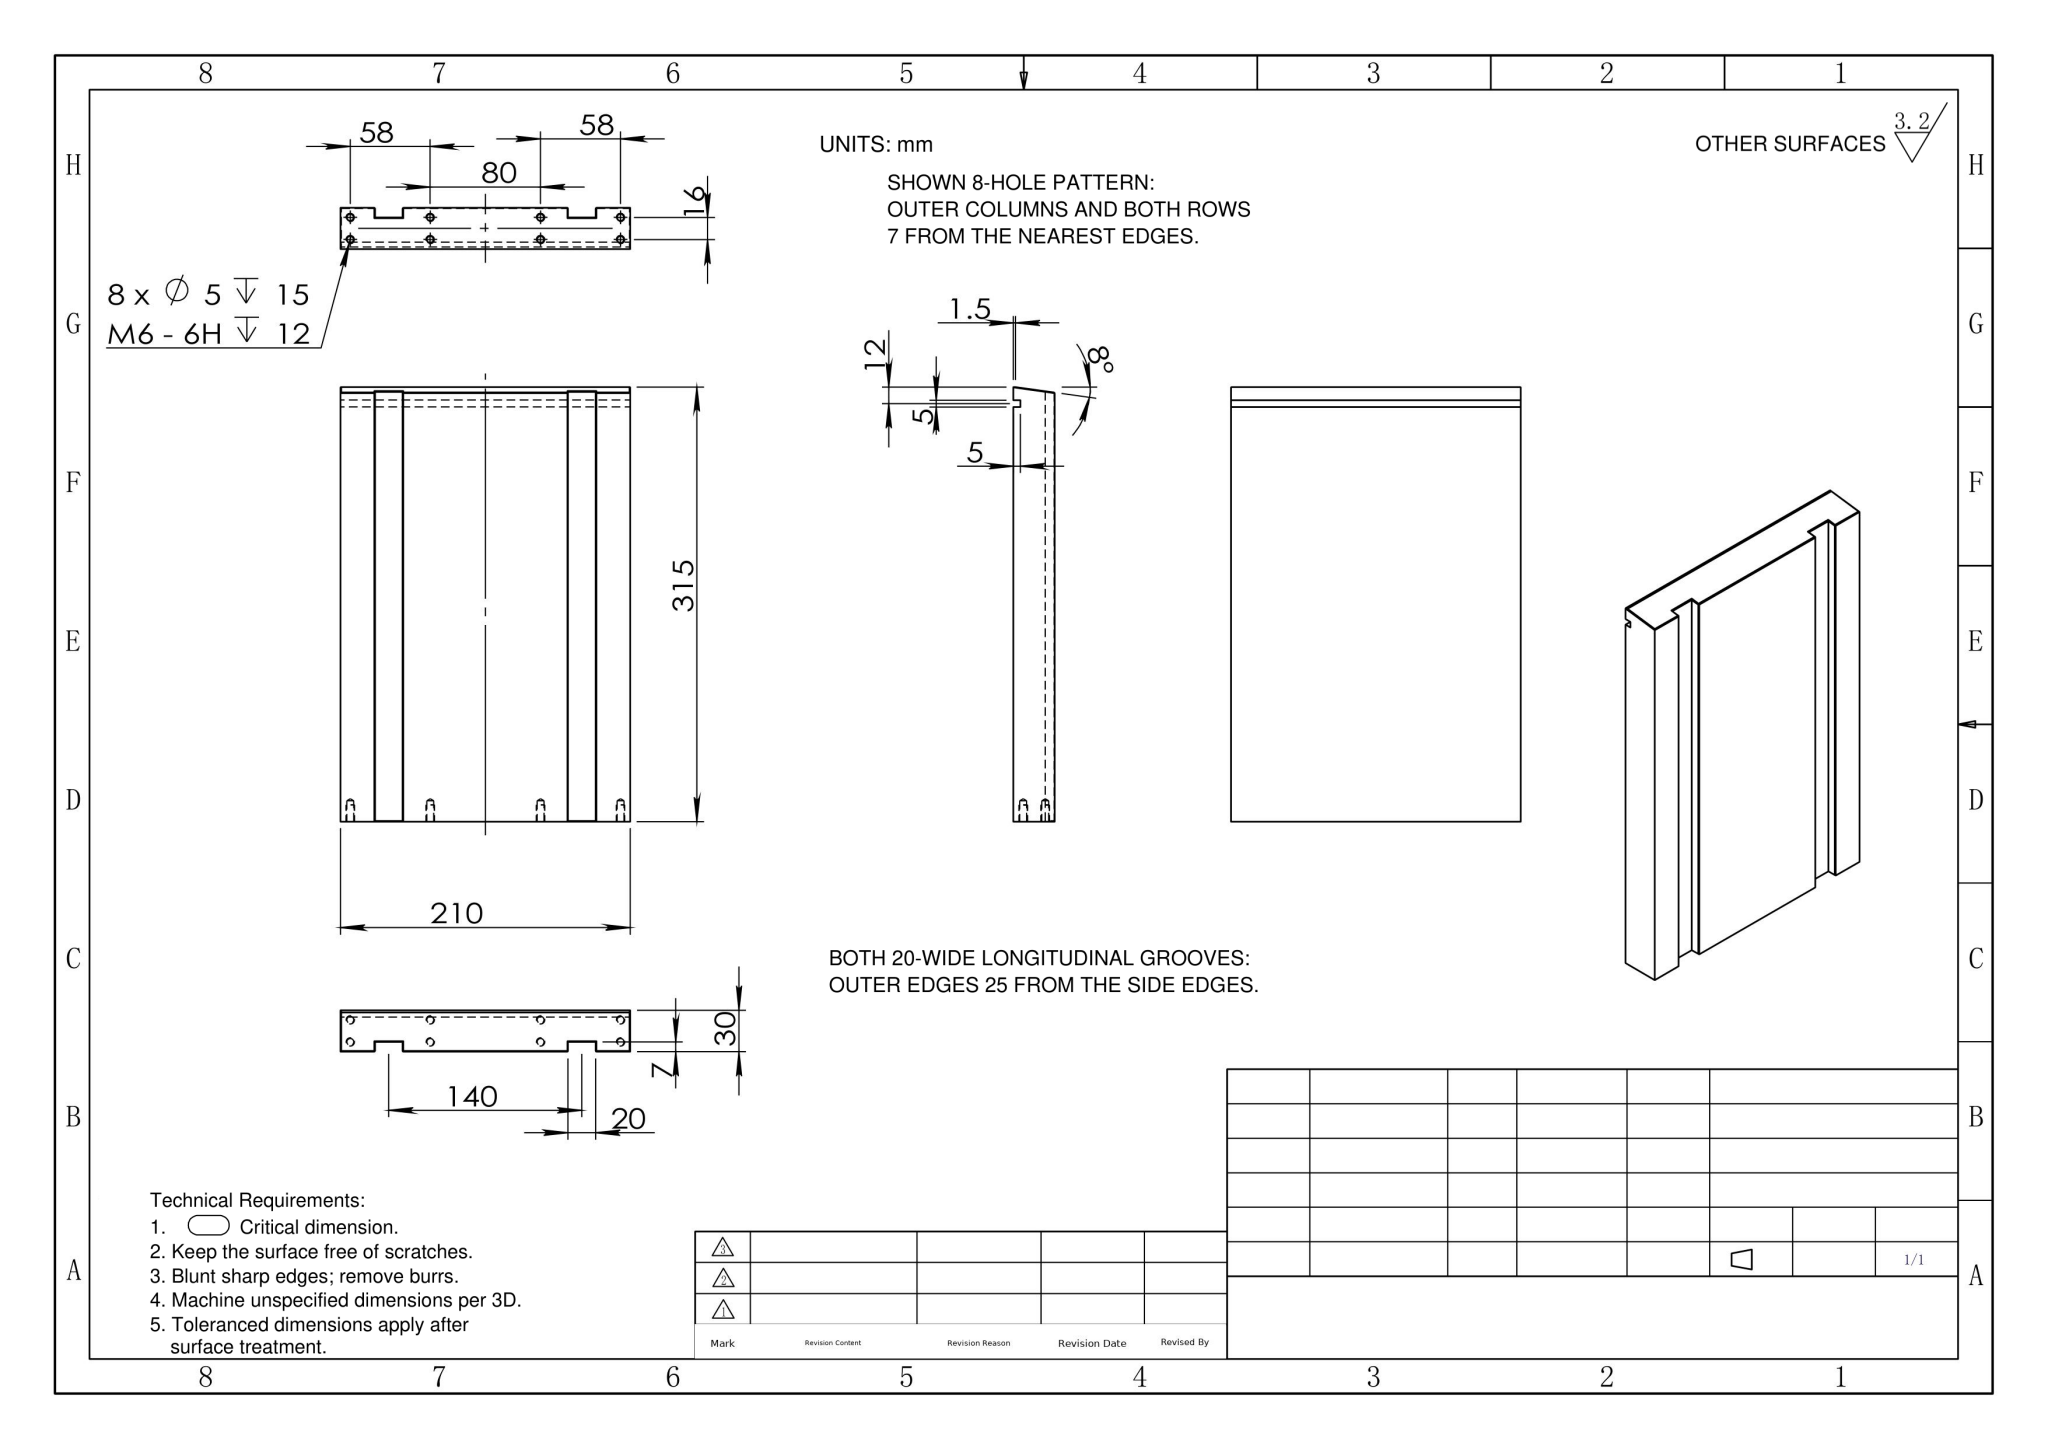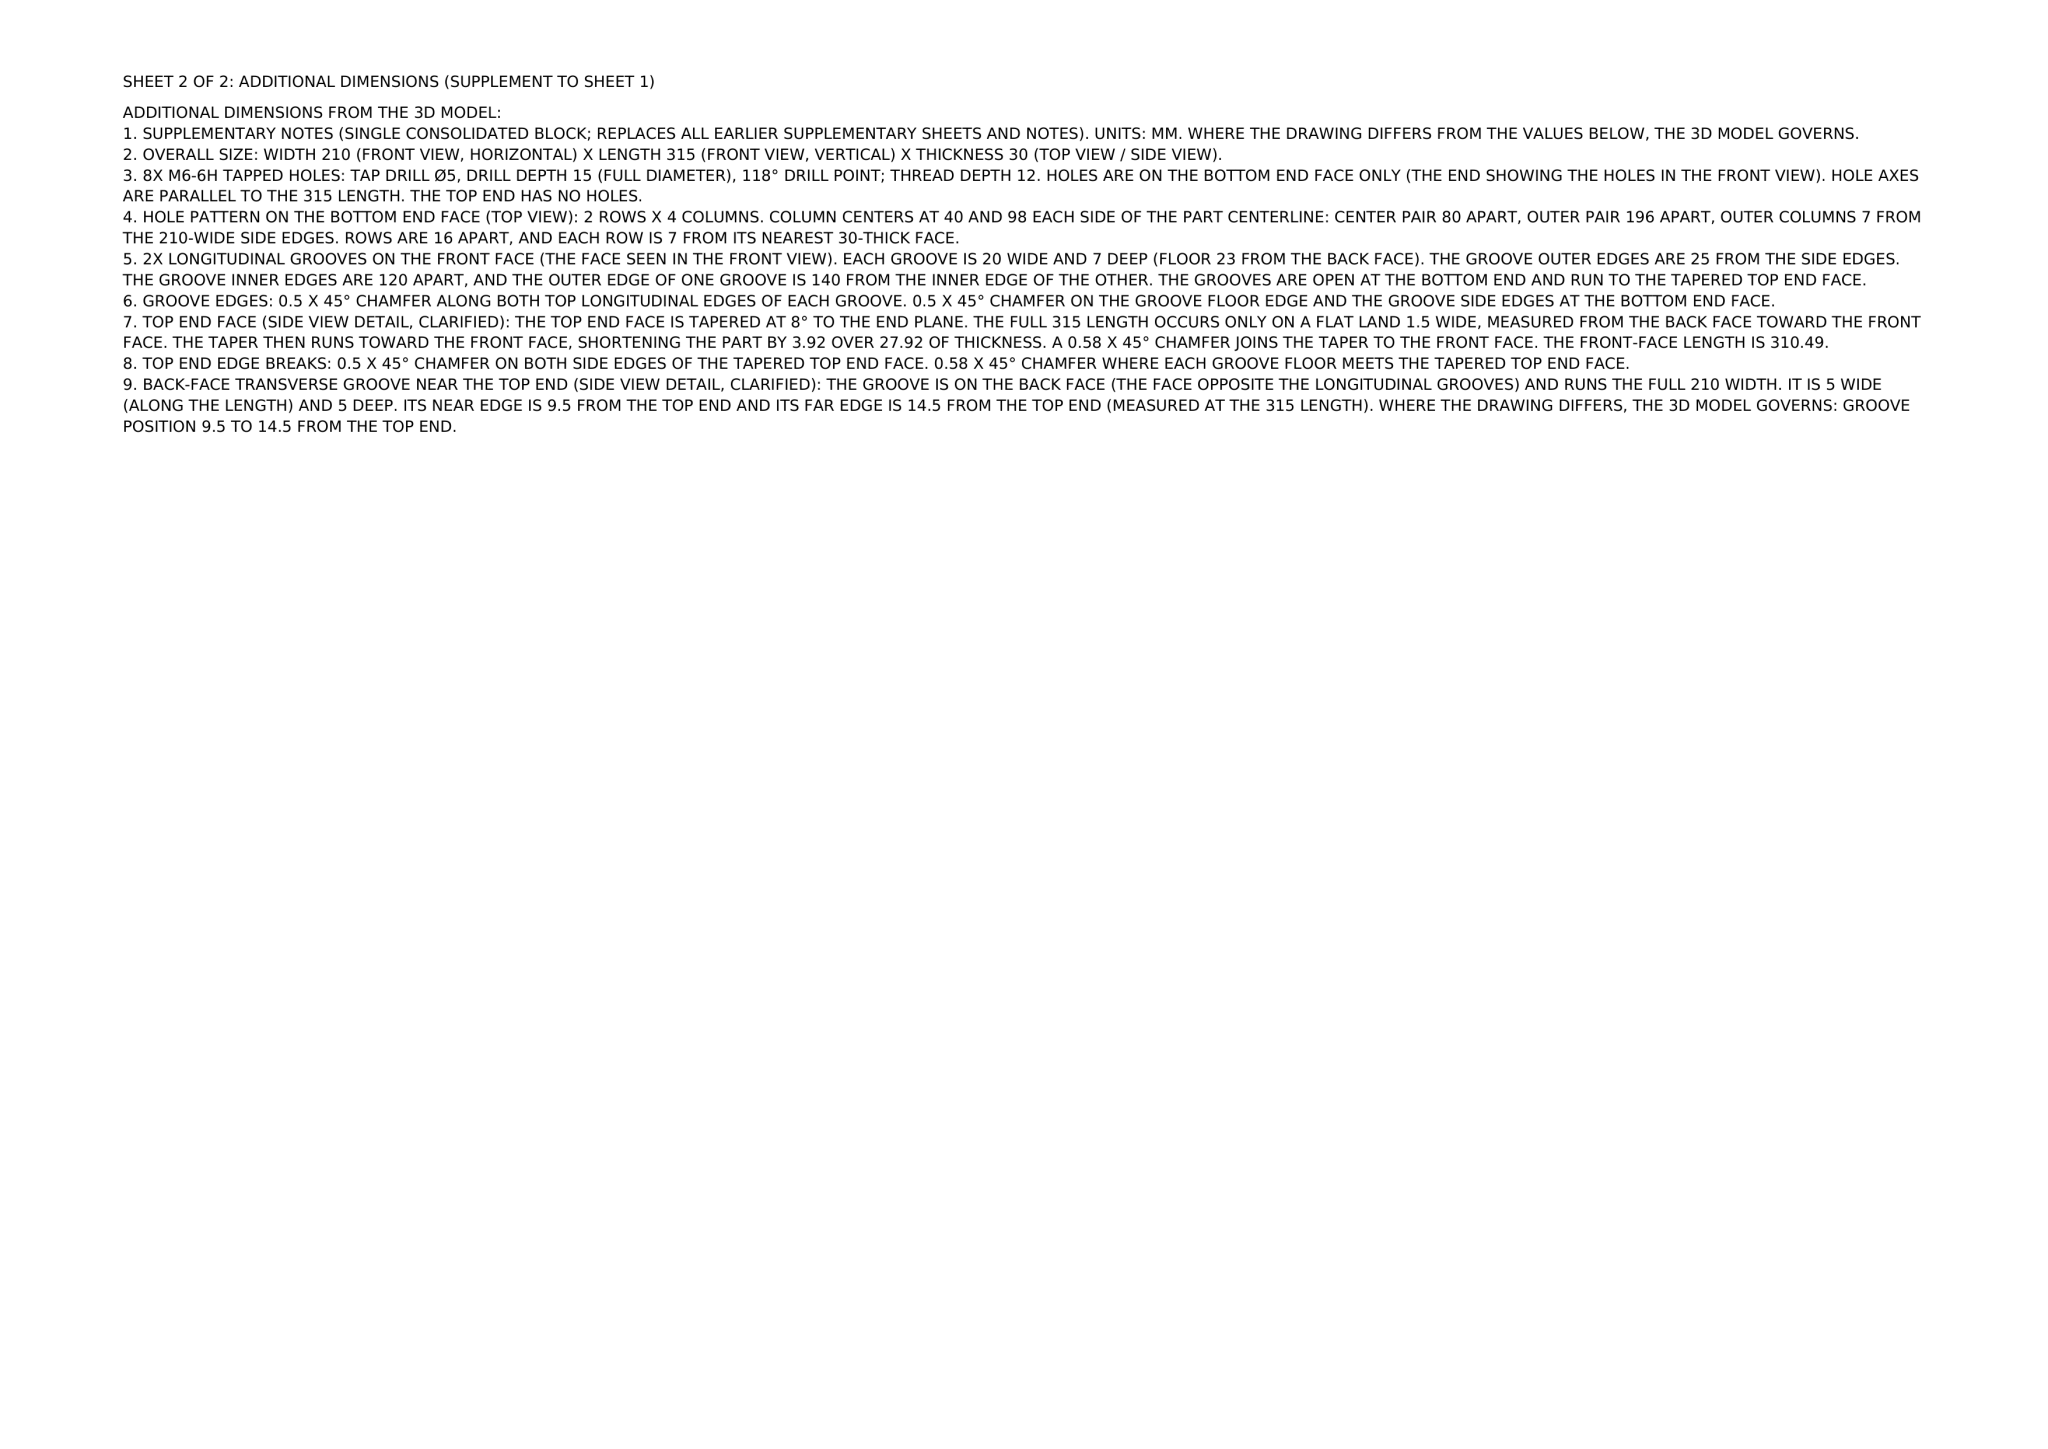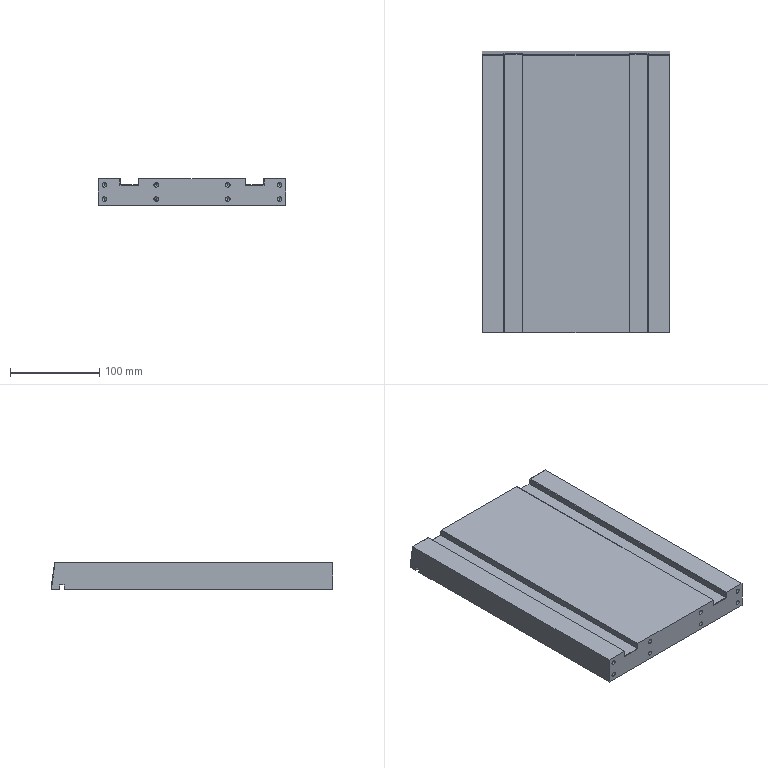Part | NX | mm | 1 solid | 72 faces | box 210 x 315 x 30 mm | volume 1877408 mm3 | plane 40 | cylinder 16 | cone 16 | commonest cylinder face diameters 5 x16